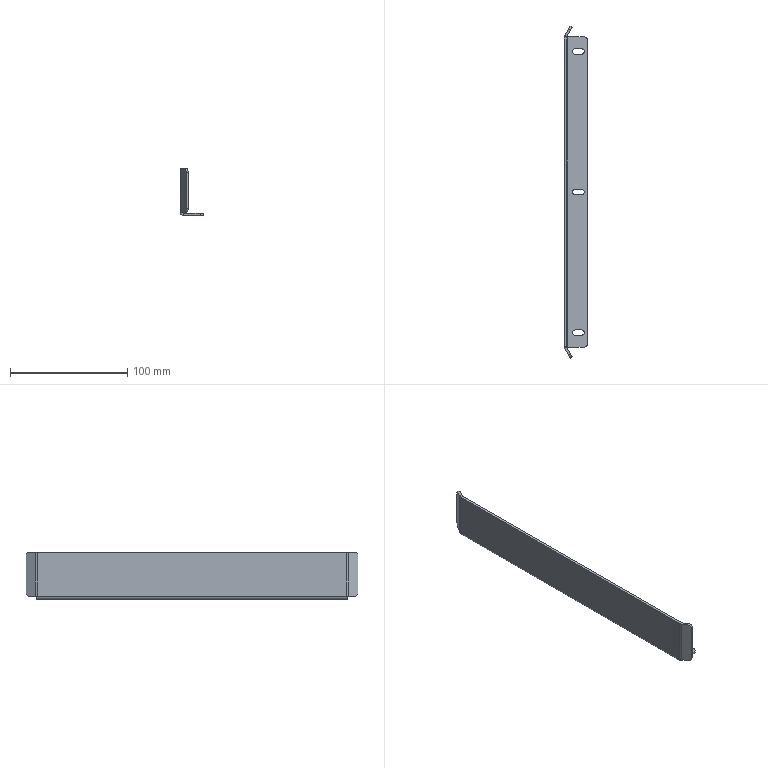Component | SolidWorks | 06-1111-3 | 1 solid | 53 faces | volume 31565 mm3 | plane 32 | cylinder 21 | commonest cylinder face diameters 4.5 x9 6 x6 5.473 x3 1.473 x3